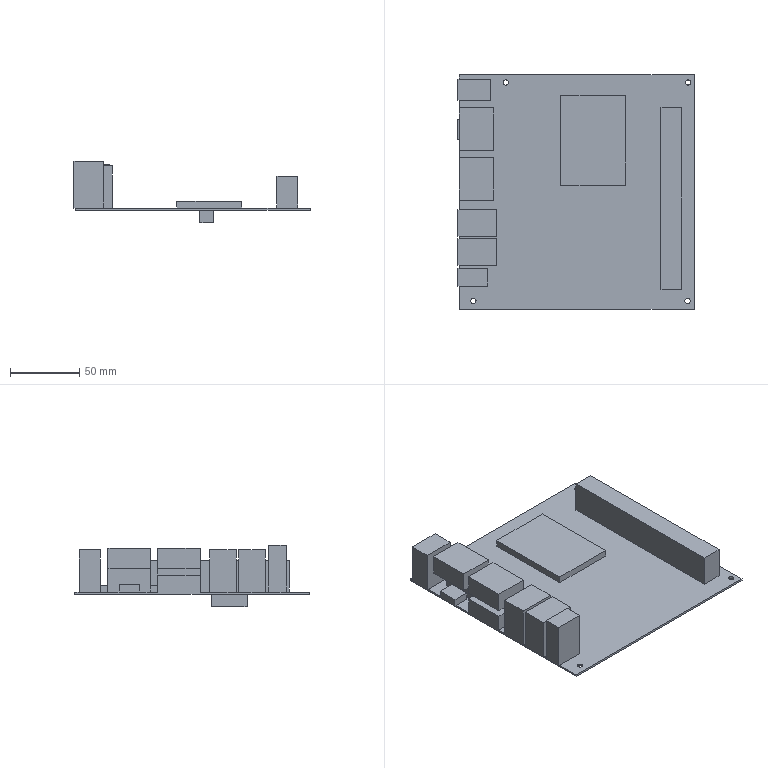Component | NX | MAIN_BOARD | 1 solid | 70 faces | volume 202125 mm3 | plane 66 | cylinder 4 | commonest cylinder face diameters 3.8 x4